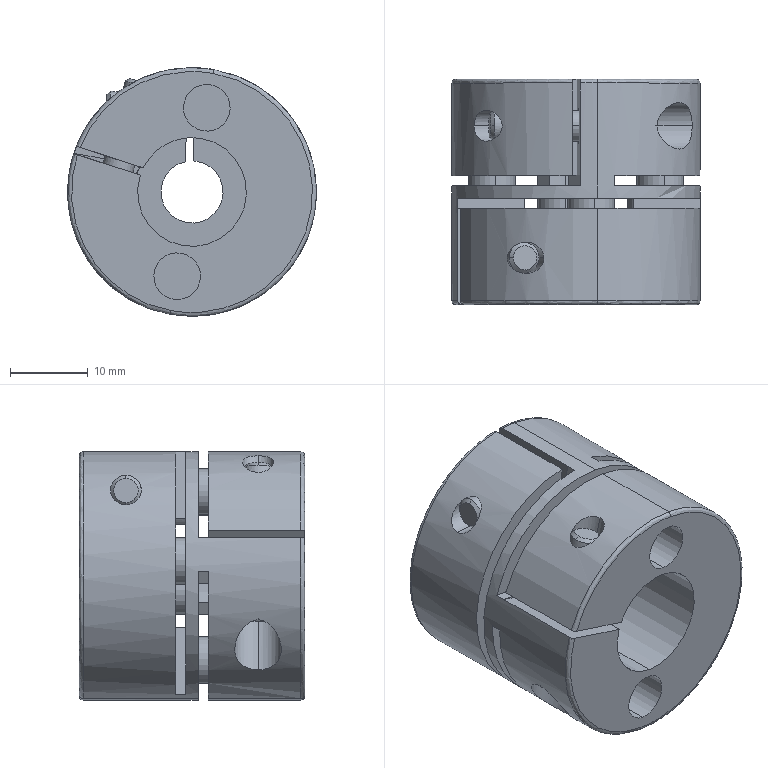Component | SolidWorks | YihadaCouplingDBA51-D32-d8-e14-1 | 1 solid | 113 faces | volume 17475 mm3 | cylinder 53 | plane 50 | spline 6 | cone 4 | commonest cylinder face diameters 6 x20 4 x10 4.5 x8 5.5 x4 32 x3 8 x3 14 x3 15 x2